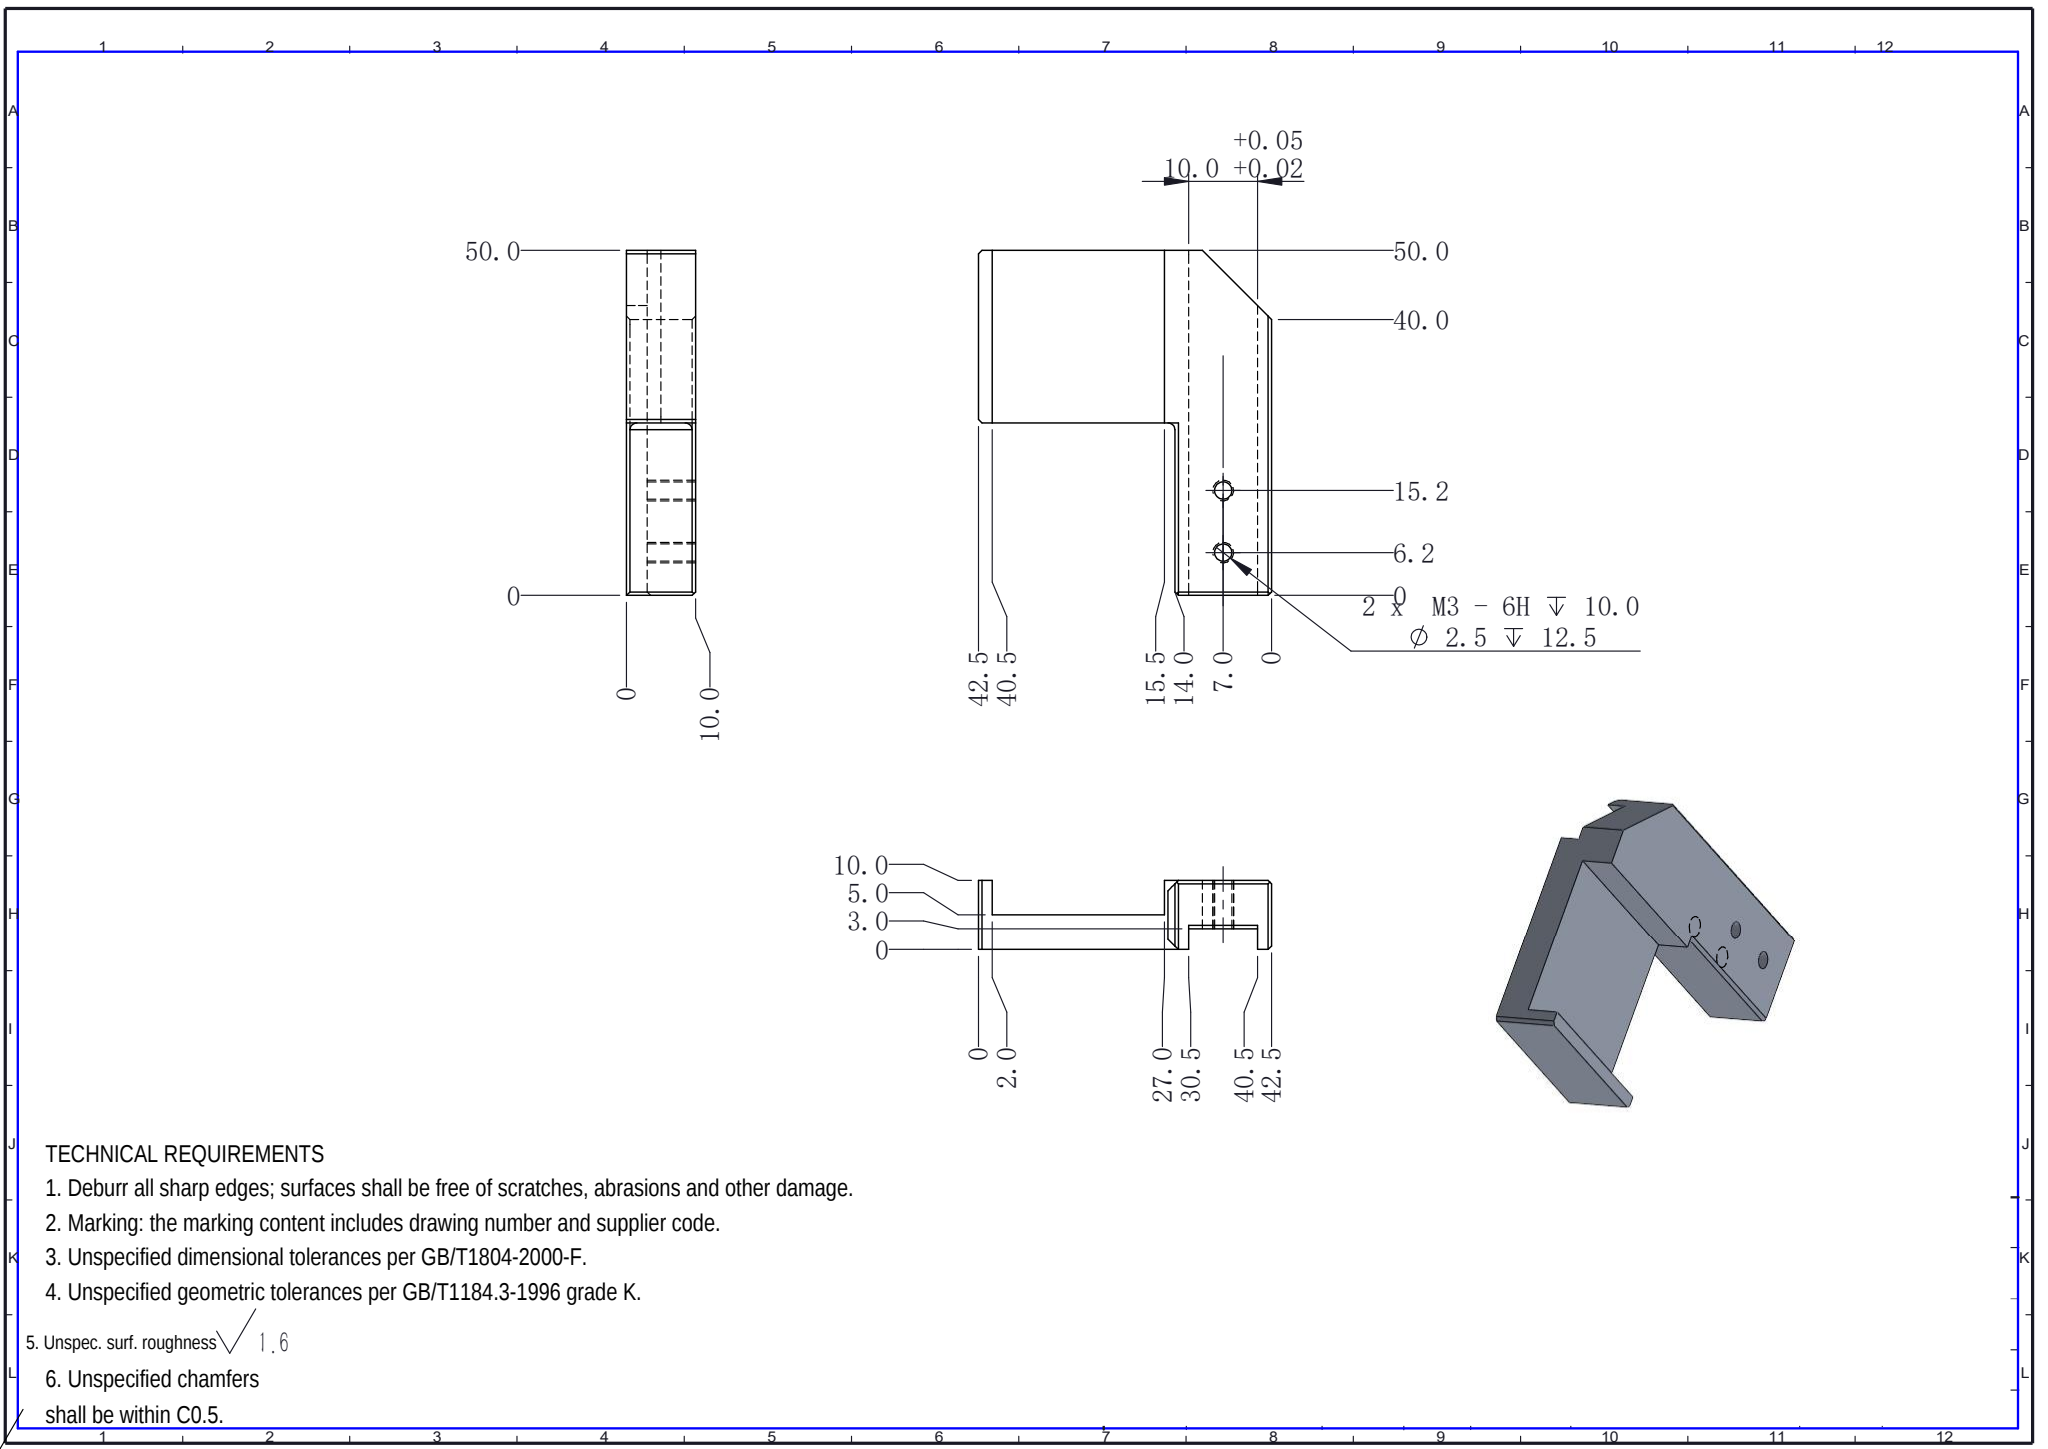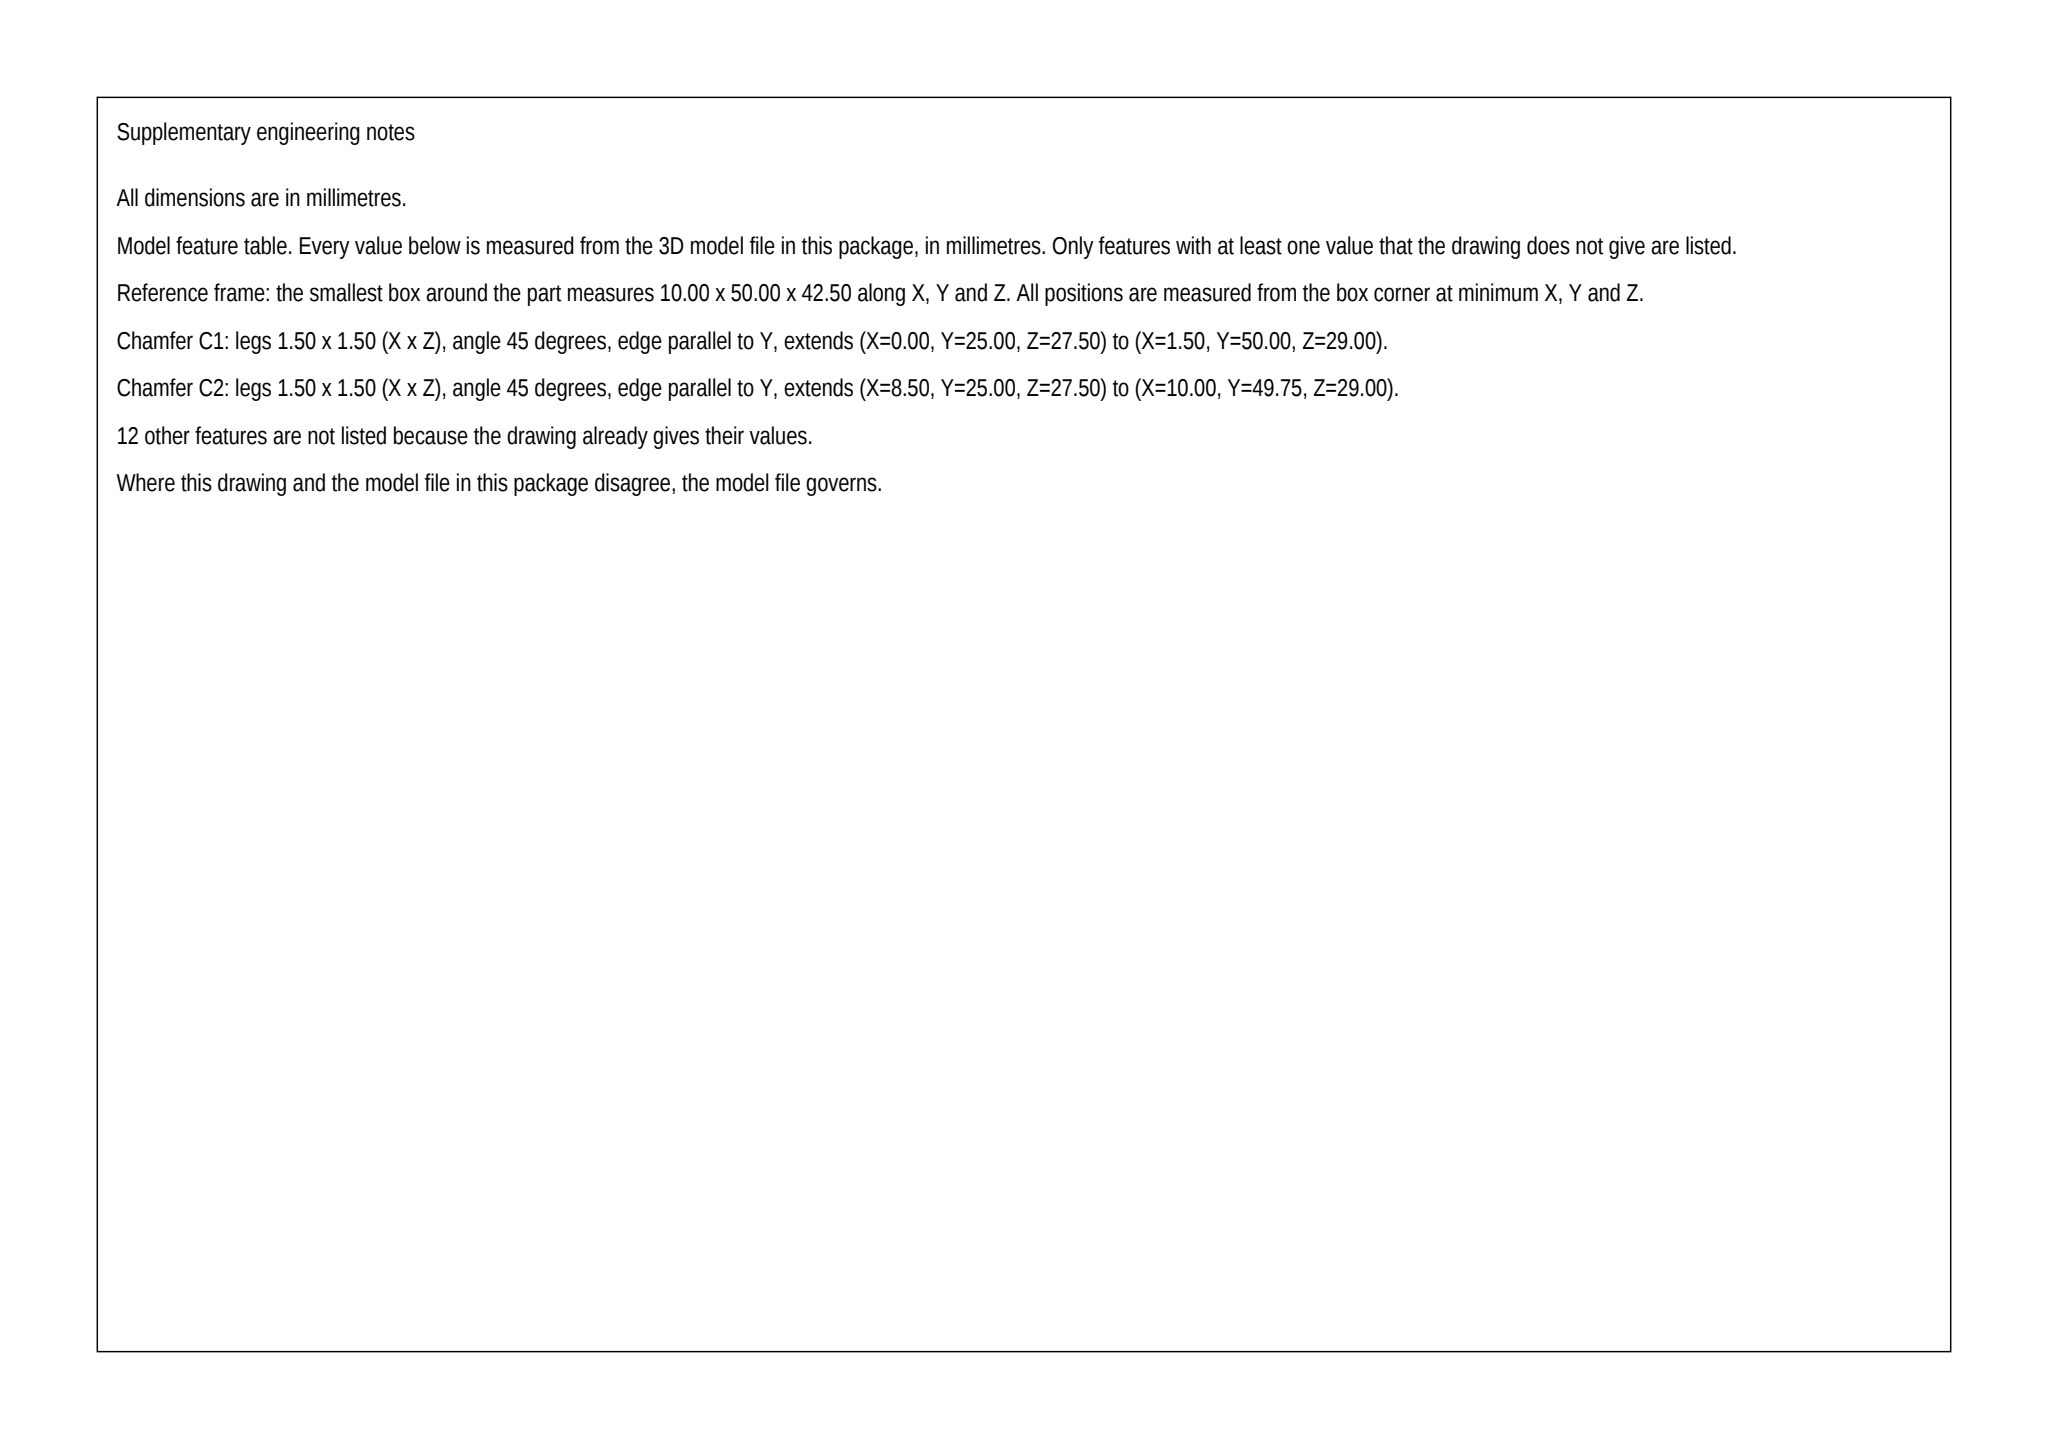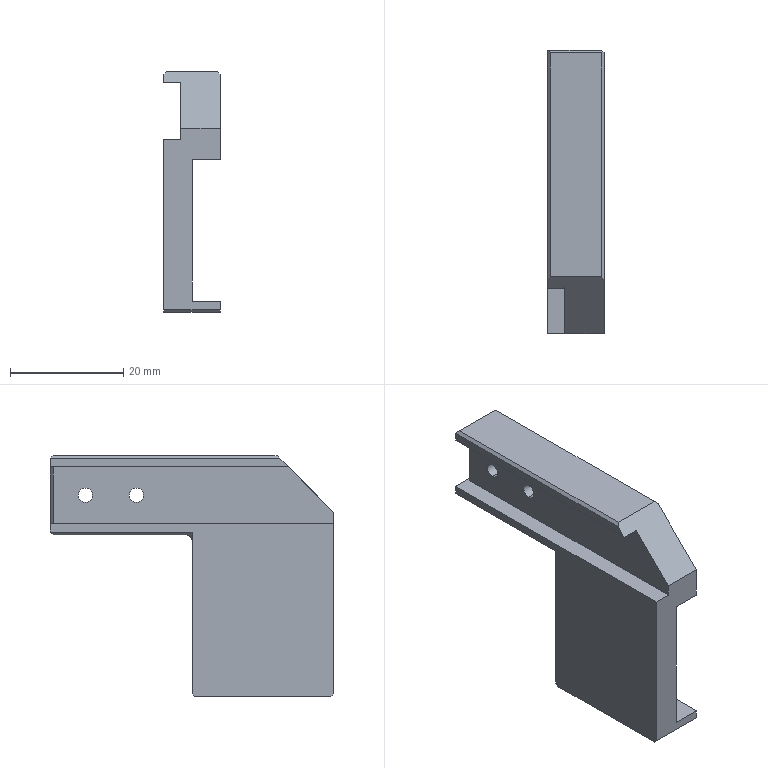Part | SolidWorks | mm | 1 solid | 32 faces | box 10 x 50 x 42.5 mm | volume 9005 mm3 | plane 27 | cylinder 5 | commonest cylinder face diameters 2.5 x4 2 x1
Drawing notes:
Ø2.0 THRU-DRILL DP 9.0 FROM 10.0 WIDE FACE, 1 PLC | from the solid: cylinder dia 2.0, axis x, length 9.0, bbox x=10.0
Ø2.0 HOLE DEPTH DP 9.0 | from the solid: cylinder [2.0,x,...,9.0]
Ø2.0 HOLE CL: 24.0 FROM 0 (BTM) x 15.0 FROM 0 (RH EDGE) | from the solid: hole at y=26.0,z=27.5; 50-26=24.0 from bottom datum, 42.5-27.5=15.0 from z=42.5 datum used by 7.0 dim on Ø2.5 holes